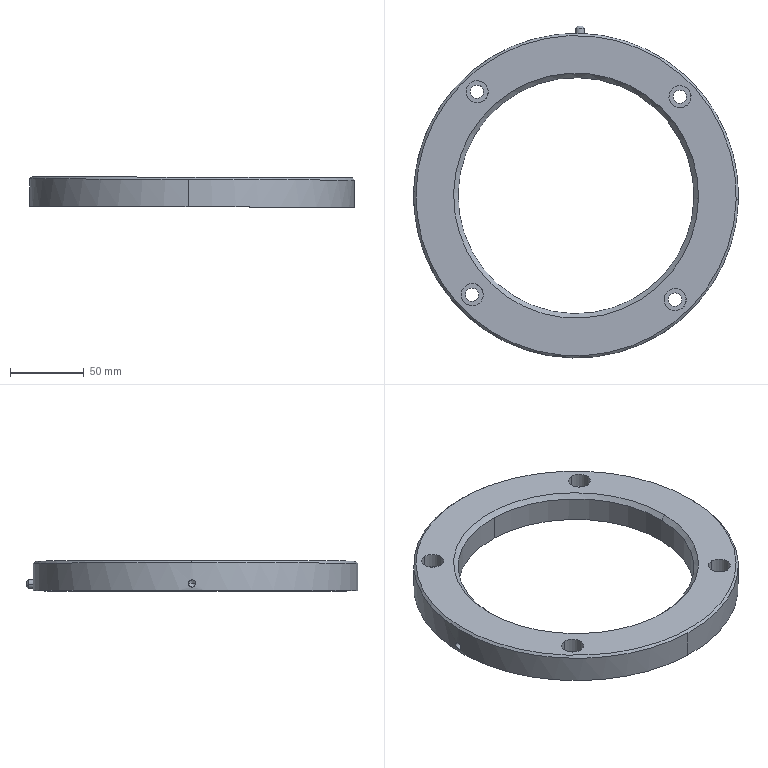Component | SolidWorks | Light-1_LightMountingPlate-1 | 1 solid | 43 faces | volume 344980 mm3 | cylinder 26 | cone 10 | plane 7 | commonest cylinder face diameters 15 x8 9 x8 5 x4 160 x2 220 x2 6 x2